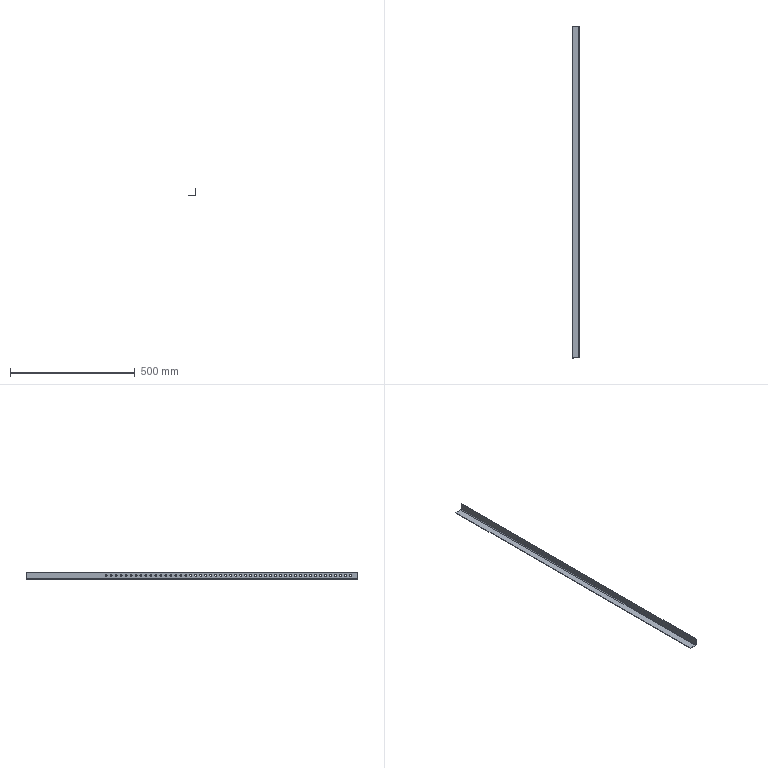Component | SolidWorks | BoxWelding-1_SupportPlate3.1-1 | 1 solid | 110 faces | box 31 x 1331 x 31 mm | volume 150123 mm3 | cylinder 102 | plane 8 | commonest cylinder face diameters 8 x100 6 x1 10 x1
build123d program:
from build123d import *

# Parameters (mm, degrees)
EXTRUDE_THIN1_DEPTH = 665.5
SKETCH2_R           = 4
CUT_EXTRUDE1_DEPTH  = 10


with BuildPart() as part:
    # Sketch1 → Extrude-Thin1 (new, symmetric)
    with BuildSketch(Plane.XY):
        with BuildLine():
            Line((-1, 30), (-1, 4))
            ThreePointArc((-1, 4), (0.4645, 0.4645), (4, -1))
            Line((4, -1), (30, -1))
            Line((30, -1), (30, 1))
            Line((30, 1), (4, 1))
            ThreePointArc((4, 1), (1.879, 1.879), (1, 4))
            Line((1, 4), (1, 30))
            Line((1, 30), (-1, 30))
        make_face()
    extrude(amount=EXTRUDE_THIN1_DEPTH, both=True)

    # Sketch2 → Cut-Extrude1 (cut)
    with BuildSketch(Plane.XZ.offset(1)):
        with Locations(Location((17, 635.5, 0), (0, 0, 270))):
            Circle(SKETCH2_R)
        with Locations(Location((17, 615.5, 0), (0, 0, 270))):
            Circle(SKETCH2_R)
        with Locations(Location((17, 595.5, 0), (0, 0, 270))):
            Circle(SKETCH2_R)
        with Locations(Location((17, 575.5, 0), (0, 0, 270))):
            Circle(SKETCH2_R)
        with Locations(Location((17, 555.5, 0), (0, 0, 270))):
            Circle(SKETCH2_R)
        with Locations(Location((17, 535.5, 0), (0, 0, 270))):
            Circle(SKETCH2_R)
        with Locations(Location((17, 515.5, 0), (0, 0, 270))):
            Circle(SKETCH2_R)
        with Locations(Location((17, 495.5, 0), (0, 0, 270))):
            Circle(SKETCH2_R)
        with Locations(Location((17, 475.5, 0), (0, 0, 270))):
            Circle(SKETCH2_R)
        with Locations(Location((17, 455.5, 0), (0, 0, 270))):
            Circle(SKETCH2_R)
        with Locations(Location((17, 435.5, 0), (0, 0, 270))):
            Circle(SKETCH2_R)
        with Locations(Location((17, 415.5, 0), (0, 0, 270))):
            Circle(SKETCH2_R)
        with Locations(Location((17, 395.5, 0), (0, 0, 270))):
            Circle(SKETCH2_R)
        with Locations(Location((17, 375.5, 0), (0, 0, 270))):
            Circle(SKETCH2_R)
        with Locations(Location((17, 355.5, 0), (0, 0, 270))):
            Circle(SKETCH2_R)
        with Locations(Location((17, 335.5, 0), (0, 0, 270))):
            Circle(SKETCH2_R)
        with Locations(Location((17, 315.5, 0), (0, 0, 270))):
            Circle(SKETCH2_R)
        with Locations(Location((17, 295.5, 0), (0, 0, 270))):
            Circle(SKETCH2_R)
        with Locations(Location((17, 275.5, 0), (0, 0, 270))):
            Circle(SKETCH2_R)
        with Locations(Location((17, 255.5, 0), (0, 0, 270))):
            Circle(SKETCH2_R)
        with Locations(Location((17, 235.5, 0), (0, 0, 270))):
            Circle(SKETCH2_R)
        with Locations(Location((17, 215.5, 0), (0, 0, 270))):
            Circle(SKETCH2_R)
        with Locations(Location((17, 195.5, 0), (0, 0, 270))):
            Circle(SKETCH2_R)
        with Locations(Location((17, 175.5, 0), (0, 0, 270))):
            Circle(SKETCH2_R)
        with Locations(Location((17, 155.5, 0), (0, 0, 270))):
            Circle(SKETCH2_R)
        with Locations(Location((17, 135.5, 0), (0, 0, 270))):
            Circle(SKETCH2_R)
        with Locations(Location((17, 115.5, 0), (0, 0, 270))):
            Circle(SKETCH2_R)
        with Locations(Location((17, 95.5, 0), (0, 0, 270))):
            Circle(SKETCH2_R)
        with Locations(Location((17, 75.5, 0), (0, 0, 270))):
            Circle(SKETCH2_R)
        with Locations(Location((17, 55.5, 0), (0, 0, 270))):
            Circle(SKETCH2_R)
        with Locations(Location((17, 35.5, 0), (0, 0, 270))):
            Circle(SKETCH2_R)
        with Locations(Location((17, 15.5, 0), (0, 0, 270))):
            Circle(SKETCH2_R)
        with Locations(Location((17, -4.5, 0), (0, 0, 270))):
            Circle(SKETCH2_R)
        with Locations(Location((17, -24.5, 0), (0, 0, 270))):
            Circle(SKETCH2_R)
        with Locations(Location((17, -44.5, 0), (0, 0, 270))):
            Circle(SKETCH2_R)
        with Locations(Location((17, -64.5, 0), (0, 0, 270))):
            Circle(SKETCH2_R)
        with Locations(Location((17, -84.5, 0), (0, 0, 270))):
            Circle(SKETCH2_R)
        with Locations(Location((17, -104.5, 0), (0, 0, 270))):
            Circle(SKETCH2_R)
        with Locations(Location((17, -124.5, 0), (0, 0, 270))):
            Circle(SKETCH2_R)
        with Locations(Location((17, -144.5, 0), (0, 0, 270))):
            Circle(SKETCH2_R)
        with Locations(Location((17, -164.5, 0), (0, 0, 270))):
            Circle(SKETCH2_R)
        with Locations(Location((17, -184.5, 0), (0, 0, 270))):
            Circle(SKETCH2_R)
        with Locations(Location((17, -204.5, 0), (0, 0, 270))):
            Circle(SKETCH2_R)
        with Locations(Location((17, -224.5, 0), (0, 0, 270))):
            Circle(SKETCH2_R)
        with Locations(Location((17, -244.5, 0), (0, 0, 270))):
            Circle(SKETCH2_R)
        with Locations(Location((17, -264.5, 0), (0, 0, 270))):
            Circle(SKETCH2_R)
        with Locations(Location((17, -284.5, 0), (0, 0, 270))):
            Circle(SKETCH2_R)
        with Locations(Location((17, -304.5, 0), (0, 0, 270))):
            Circle(SKETCH2_R)
        with Locations(Location((17, -324.5, 0), (0, 0, 270))):
            Circle(SKETCH2_R)
        with Locations(Location((17, -344.5, 0), (0, 0, 270))):
            Circle(SKETCH2_R)
    extrude(amount=-CUT_EXTRUDE1_DEPTH, mode=Mode.SUBTRACT)


solid = part.part

# Placed as in the assembly
solid = solid.moved(Location((270.622, 621.001, -188.987), (90, 0, 90)))